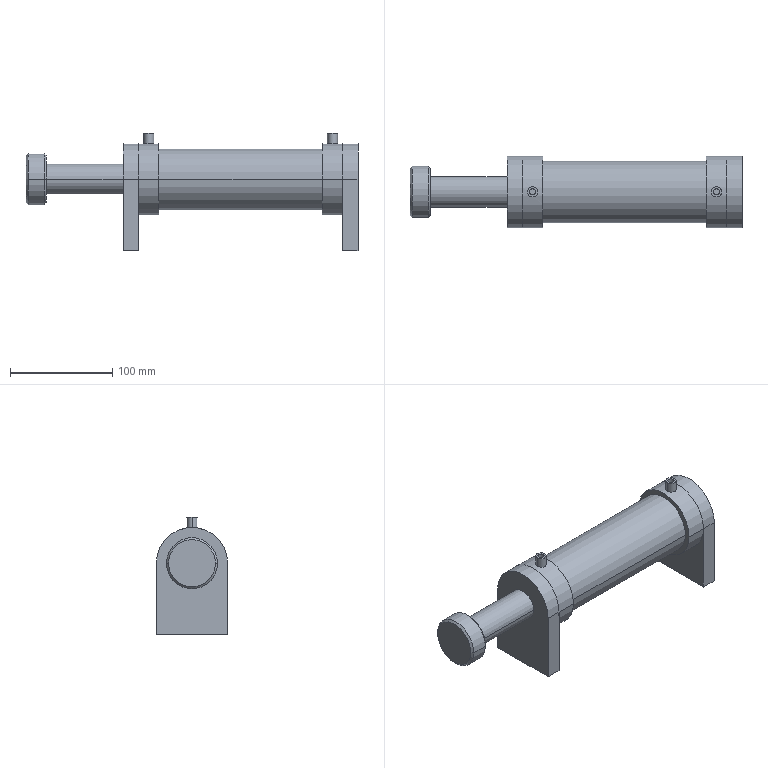Component | SolidWorks | HydraulicCylinderC-1 | 5 solids | 54 faces | box 325 x 70 x 115 mm | volume 891163 mm3 | cylinder 28 | plane 22 | cone 4 | commonest cylinder face diameters 10 x8 30 x6 70 x6 6 x4 50 x2 60 x2 | material 45
build123d program:
from build123d import *

# Parameters (mm, degrees)
SKETCH2_2_R           = 25
BOSS_EXTRUDE1_DEPTH   = 20
CHAMFER1_SIZE         = 2
SKETCH3_R             = 15
BOSS_EXTRUDE2_DEPTH   = 15
SKETCH2_R             = 5
CUT_EXTRUDE2_DEPTH    = 40
SKETCH4_R             = 5
SKETCH4_R_2           = 3
BOSS_EXTRUDE3_DEPTH   = 45
BOSS_EXTRUDE3_2_DEPTH = 45


with BuildPart() as part:
    # Sketch1 → Revolve1 (revolve)
    with BuildSketch(Plane.XY, mode=Mode.PRIVATE) as revolve1_sk:
        Polygon((0, 0), (0, 15), (90, 15), (90, 35), (110, 35), (110, 30), (270, 30), (270, 35), (290, 35), (290, 0), align=None)
    revolve(revolve1_sk.sketch.rotate(Axis((0, 0, 0), (1, 0, 0)), 180), axis=Axis((0, 0, 0), (1, 0, 0)))

    # Sketch2_2 → Boss-Extrude1 (add)
    with BuildSketch(Plane.ZY):
        with Locations(Location((0, 0, 0), (0, 0, 270))):
            Circle(SKETCH2_2_R)
    extrude(amount=BOSS_EXTRUDE1_DEPTH)

    # Chamfer1
    chamfer1_edges = [part.edges().sort_by_distance(p)[0] for p in [
        (0, 25, 0),
        (-20, 25, 0),
    ]]
    chamfer(chamfer1_edges, length=CHAMFER1_SIZE)

    # Sketch2 → Cut-Extrude2 (cut)
    with BuildSketch(Plane.XY):
        with Locations(Location((100, 0, 0), (0, 0, 180))):
            Circle(SKETCH2_R)
        with Locations(Location((280, 0, 0), (0, 0, 180))):
            Circle(SKETCH2_R)
    extrude(amount=CUT_EXTRUDE2_DEPTH, mode=Mode.SUBTRACT)


with BuildPart() as body_2:
    # Sketch3 → Boss-Extrude2 (new body)
    with BuildSketch(Plane.ZY.offset(-90)):
        with BuildLine():
            Line((0, 35), (-70, 35))
            Line((-70, 35), (-70, -35))
            Line((-70, -35), (0, -35))
            ThreePointArc((0, -35), (35, 0), (0, 35))
        make_face()
        with Locations(Location((0, 0, 0), (0, 0, 270))):
            Circle(SKETCH3_R, mode=Mode.SUBTRACT)
    extrude(amount=BOSS_EXTRUDE2_DEPTH)


with BuildPart() as body_3:
    # Mirror1: mirrored copy
    add(body_2.part.mirror(Plane.ZY.offset(-190)))


with BuildPart() as body_4:
    # Sketch4 → Boss-Extrude3 (new body)
    with BuildSketch(Plane.XY):
        with Locations(Location((100, 0, 0), (0, 0, 180))):
            Circle(SKETCH4_R)
        with Locations(Location((100, 0, 0), (0, 0, 180))):
            Circle(SKETCH4_R_2, mode=Mode.SUBTRACT)
    extrude(amount=BOSS_EXTRUDE3_DEPTH)


with BuildPart() as body_5:
    # Sketch4 → Boss-Extrude3 2 (new body)
    with BuildSketch(Plane.XY):
        with Locations(Location((280, 0, 0), (0, 0, 180))):
            Circle(SKETCH4_R)
        with Locations(Location((280, 0, 0), (0, 0, 180))):
            Circle(SKETCH4_R_2, mode=Mode.SUBTRACT)
    extrude(amount=BOSS_EXTRUDE3_2_DEPTH)


solid = Compound([part.part, body_2.part, body_3.part, body_4.part, body_5.part])

# Placed as in the assembly
solid = solid.moved(Location((14.187, 248.429, 822.267), (0, 0, 0)))